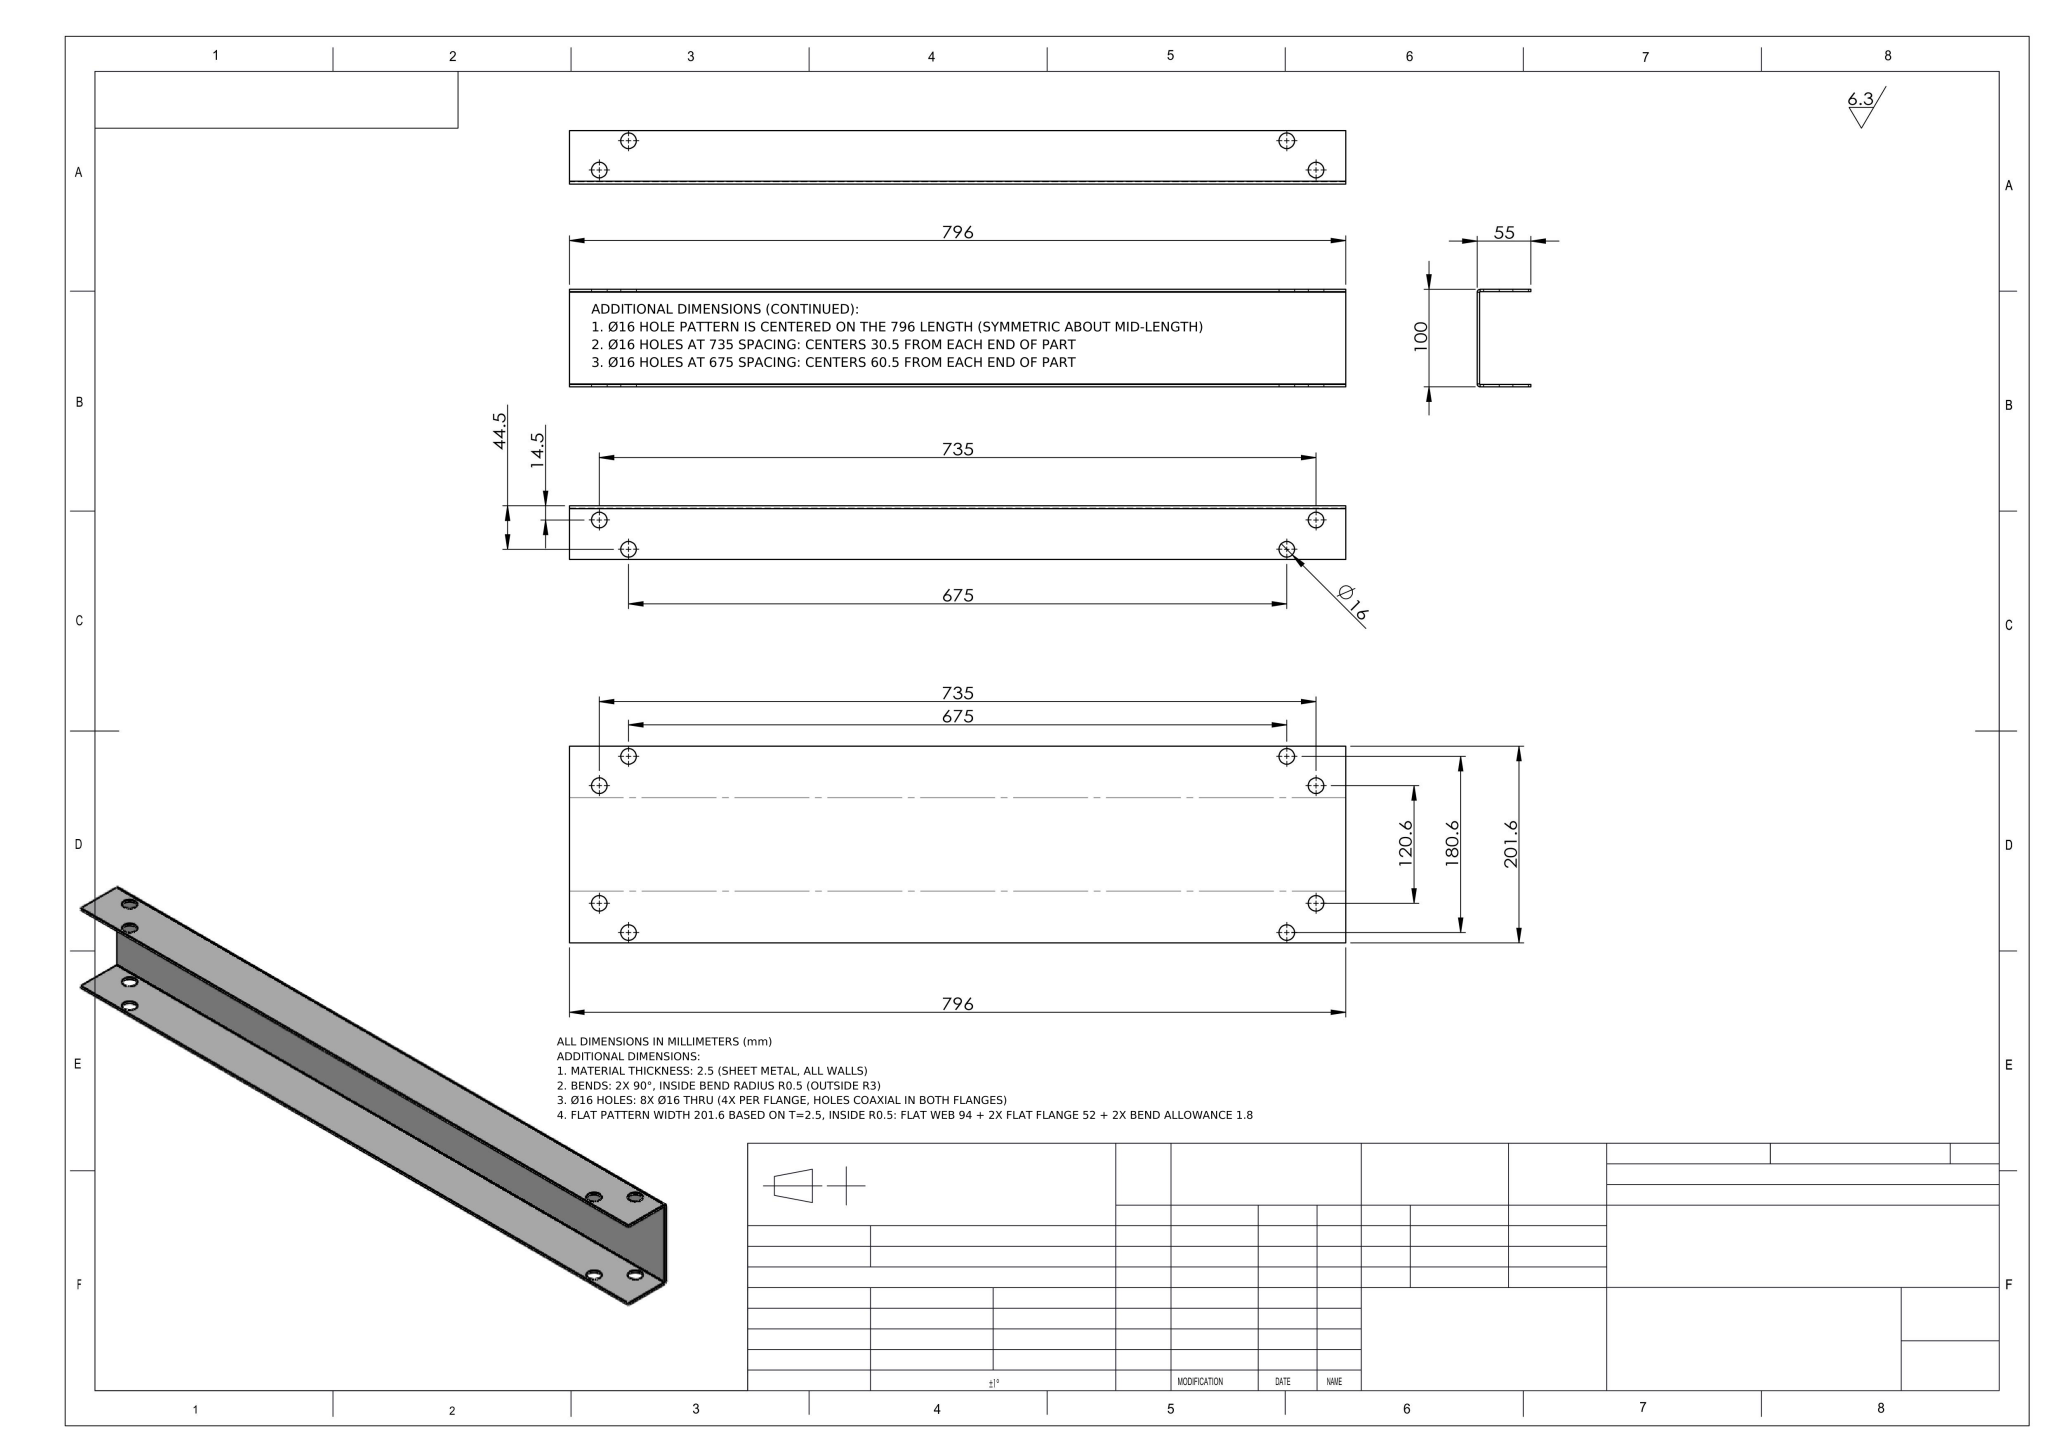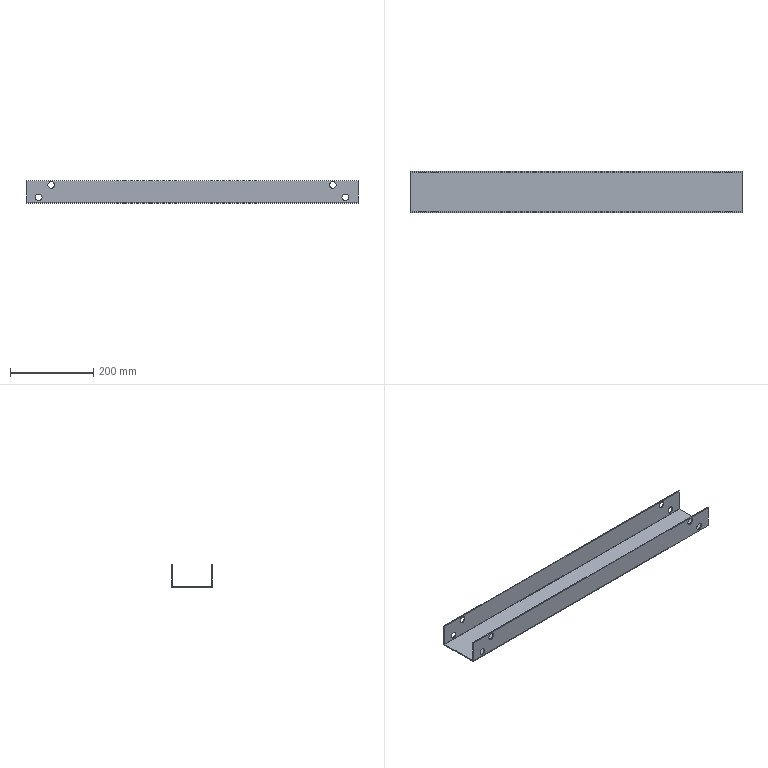Part | NX | mm | 1 solid | 38 faces | box 796 x 100 x 55 mm | volume 400939 mm3 | cylinder 20 | plane 18 | commonest cylinder face diameters 16 x16 6 x2 1 x2